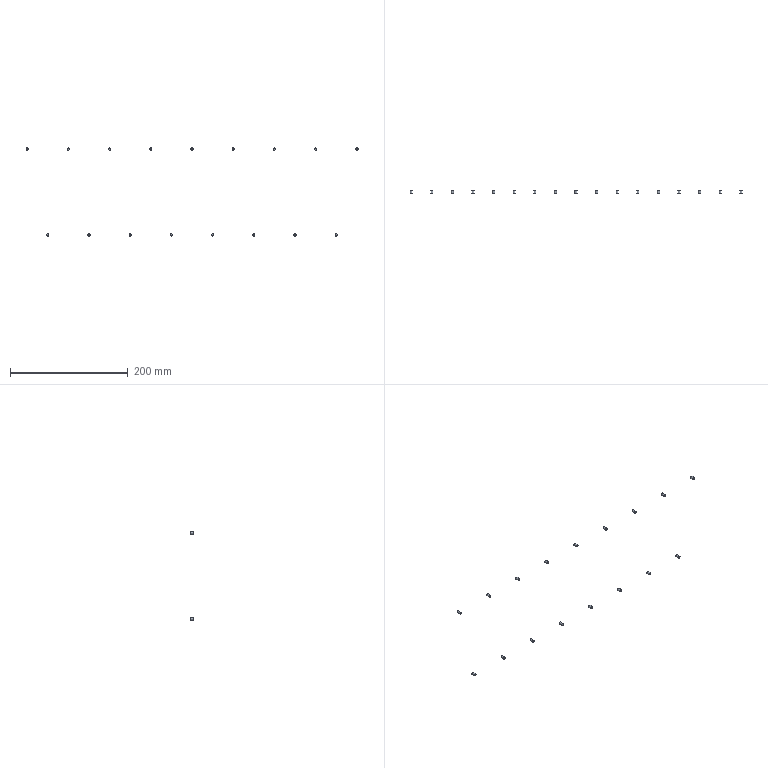Component | NX | PIN | 17 solids | 51 faces | volume 1282 mm3 | plane 34 | cylinder 17 | commonest cylinder face diameters 4 x17